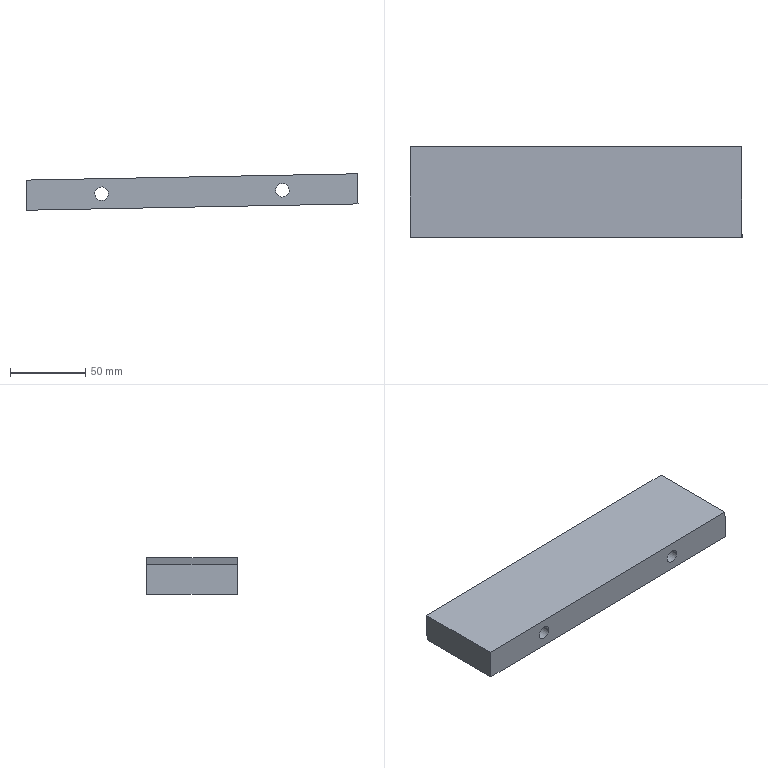Component | SolidWorks | 12TopPostMountingPlateSpacer-1 | 1 solid | 24 faces | box 220.34 x 60 x 24.19 mm | volume 248965 mm3 | cylinder 12 | plane 8 | cone 4 | commonest cylinder face diameters 15 x4 9 x4 8.5 x4 | material A3 Steel
build123d program:
from build123d import *

# Parameters (mm, degrees)
SKETCH1_W                                          = 220
SKETCH1_H                                          = 20
BOSS_EXTRUDE1_DEPTH                                = 30
M10_TAPPED_HOLE1_D                                 = 8.5
M10_TAPPED_HOLE1_DEPTH                             = 24.5
M10_TAPPED_HOLE1_TIP                               = 2.554
HOLE_SIZE_ACCORDING_TO_TYPE_1_OF_HEXAG_D           = 9
HOLE_SIZE_ACCORDING_TO_TYPE_1_OF_HEXAG_CBORE_D     = 15
HOLE_SIZE_ACCORDING_TO_TYPE_1_OF_HEXAG_CBORE_DEPTH = 20


with BuildPart() as part:
    # Sketch1 → Boss-Extrude1 (new, symmetric)
    with BuildSketch(Plane.XY):
        Rectangle(SKETCH1_W, SKETCH1_H)
    extrude(amount=BOSS_EXTRUDE1_DEPTH, both=True)

    # M10 Tapped Hole1
    with Locations(Plane(origin=(-90, 0, -30), x_dir=(-1, 0, 0), z_dir=(0, 0, -1))):
        with Locations((0, 0), (-180, 0)):
            Hole(M10_TAPPED_HOLE1_D / 2, depth=M10_TAPPED_HOLE1_DEPTH)
            with Locations((0, 0, -(M10_TAPPED_HOLE1_DEPTH + M10_TAPPED_HOLE1_TIP / 2))):  # 118° drill point
                Cone(0, M10_TAPPED_HOLE1_D / 2, M10_TAPPED_HOLE1_TIP, mode=Mode.SUBTRACT)

    # Hole Size _According to_ Type 1 of Hexag (through all)
    with Locations(Plane(origin=(60, 0, -30), x_dir=(-1, 0, 0), z_dir=(0, 0, -1))):
        with Locations((0, 0), (120, 0)):
            CounterBoreHole(HOLE_SIZE_ACCORDING_TO_TYPE_1_OF_HEXAG_D / 2, HOLE_SIZE_ACCORDING_TO_TYPE_1_OF_HEXAG_CBORE_D / 2, HOLE_SIZE_ACCORDING_TO_TYPE_1_OF_HEXAG_CBORE_DEPTH)


solid = part.part

# Placed as in the assembly
solid = solid.moved(Location((1158.199, -1865.522, 2192.697), (90, 0, 1.091)))
STEP:
#1=COLOUR_RGB('',0.7922,0.8196,0.9333);
#2=FILL_AREA_STYLE_COLOUR('',#1);
#3=FILL_AREA_STYLE('',(#2));
#4=SURFACE_STYLE_FILL_AREA(#3);
#5=SURFACE_SIDE_STYLE('',(#4));
#6=SURFACE_STYLE_USAGE(.BOTH.,#5);
#7=PRESENTATION_STYLE_ASSIGNMENT((#6));
#8=CARTESIAN_POINT('',(48.255,-73.052,86.377));
#9=VERTEX_POINT('',#8);
#10=CARTESIAN_POINT('',(47.665,-73.052,86.366));
#11=VERTEX_POINT('',#10);
#12=CARTESIAN_POINT('',(47.96,-73.052,86.372));
#13=DIRECTION('',(-0.,1.,-0.));
#14=DIRECTION('',(-0.9998,0.,-0.01904));
#15=AXIS2_PLACEMENT_3D('',#12,#13,#14);
#16=CIRCLE('',#15,0.2953);
#17=EDGE_CURVE('',#9,#11,#16,.T.);
#18=ORIENTED_EDGE('',*,*,#17,.F.);
#19=CARTESIAN_POINT('',(48.255,-72.265,86.377));
#20=VERTEX_POINT('',#19);
#21=CARTESIAN_POINT('',(48.255,-72.265,86.377));
#22=DIRECTION('',(-0.,1.,-0.));
#23=VECTOR('',#22,39.37);
#24=LINE('',#21,#23);
#25=EDGE_CURVE('',#9,#20,#24,.T.);
#26=ORIENTED_EDGE('',*,*,#25,.T.);
#27=CARTESIAN_POINT('',(47.665,-72.265,86.366));
#28=VERTEX_POINT('',#27);
#29=CARTESIAN_POINT('',(47.96,-72.265,86.372));
#30=DIRECTION('',(-0.,1.,-0.));
#31=DIRECTION('',(-0.9998,0.,-0.01904));
#32=AXIS2_PLACEMENT_3D('',#29,#30,#31);
#33=CIRCLE('',#32,0.2953);
#34=EDGE_CURVE('',#20,#28,#33,.T.);
#35=ORIENTED_EDGE('',*,*,#34,.T.);
#36=CARTESIAN_POINT('',(47.665,-72.265,86.366));
#37=DIRECTION('',(-0.,1.,-0.));
#38=VECTOR('',#37,39.37);
#39=LINE('',#36,#38);
#40=EDGE_CURVE('',#11,#28,#39,.T.);
#41=ORIENTED_EDGE('',*,*,#40,.F.);
#42=EDGE_LOOP('',(#18,#26,#35,#41));
#43=FACE_OUTER_BOUND('',#42,.T.);
#44=CARTESIAN_POINT('',(47.96,-72.265,86.372));
#45=DIRECTION('',(-0.,1.,-0.));
#46=DIRECTION('',(-0.9998,0.,-0.01904));
#47=AXIS2_PLACEMENT_3D('',#44,#45,#46);
#48=CYLINDRICAL_SURFACE('',#47,0.2953);
#49=ADVANCED_FACE('',(#43),#48,.F.);
#50=CARTESIAN_POINT('',(48.137,-74.627,86.375));
#51=VERTEX_POINT('',#50);
#52=CARTESIAN_POINT('',(47.783,-74.627,86.368));
#53=VERTEX_POINT('',#52);
#54=CARTESIAN_POINT('',(47.96,-74.627,86.372));
#55=DIRECTION('',(-0.,1.,-0.));
#56=DIRECTION('',(-0.9998,0.,-0.01904));
#57=AXIS2_PLACEMENT_3D('',#54,#55,#56);
#58=CIRCLE('',#57,0.1772);
#59=EDGE_CURVE('',#51,#53,#58,.T.);
#60=ORIENTED_EDGE('',*,*,#59,.F.);
#61=CARTESIAN_POINT('',(48.137,-73.052,86.375));
#62=VERTEX_POINT('',#61);
#63=CARTESIAN_POINT('',(48.137,-72.265,86.375));
#64=DIRECTION('',(-0.,1.,-0.));
#65=VECTOR('',#64,39.37);
#66=LINE('',#63,#65);
#67=EDGE_CURVE('',#51,#62,#66,.T.);
#68=ORIENTED_EDGE('',*,*,#67,.T.);
#69=CARTESIAN_POINT('',(47.783,-73.052,86.368));
#70=VERTEX_POINT('',#69);
#71=CARTESIAN_POINT('',(47.96,-73.052,86.372));
#72=DIRECTION('',(-0.,1.,-0.));
#73=DIRECTION('',(-0.9998,0.,-0.01904));
#74=AXIS2_PLACEMENT_3D('',#71,#72,#73);
#75=CIRCLE('',#74,0.1772);
#76=EDGE_CURVE('',#62,#70,#75,.T.);
#77=ORIENTED_EDGE('',*,*,#76,.T.);
#78=CARTESIAN_POINT('',(47.783,-72.265,86.368));
#79=DIRECTION('',(-0.,1.,-0.));
#80=VECTOR('',#79,39.37);
#81=LINE('',#78,#80);
#82=EDGE_CURVE('',#53,#70,#81,.T.);
#83=ORIENTED_EDGE('',*,*,#82,.F.);
#84=EDGE_LOOP('',(#60,#68,#77,#83));
#85=FACE_OUTER_BOUND('',#84,.T.);
#86=CARTESIAN_POINT('',(47.96,-72.265,86.372));
#87=DIRECTION('',(-0.,1.,-0.));
#88=DIRECTION('',(-0.9998,0.,-0.01904));
#89=AXIS2_PLACEMENT_3D('',#86,#87,#88);
#90=CYLINDRICAL_SURFACE('',#89,0.1772);
#91=ADVANCED_FACE('',(#85),#90,.F.);
#92=CARTESIAN_POINT('',(43.532,-73.052,86.287));
#93=VERTEX_POINT('',#92);
#94=CARTESIAN_POINT('',(42.941,-73.052,86.276));
#95=VERTEX_POINT('',#94);
#96=CARTESIAN_POINT('',(43.237,-73.052,86.282));
#97=DIRECTION('',(-0.,1.,-0.));
#98=DIRECTION('',(-0.9998,0.,-0.01904));
#99=AXIS2_PLACEMENT_3D('',#96,#97,#98);
#100=CIRCLE('',#99,0.2953);
#101=EDGE_CURVE('',#93,#95,#100,.T.);
#102=ORIENTED_EDGE('',*,*,#101,.F.);
#103=CARTESIAN_POINT('',(43.532,-72.265,86.287));
#104=VERTEX_POINT('',#103);
#105=CARTESIAN_POINT('',(43.532,-72.265,86.287));
#106=DIRECTION('',(-0.,1.,-0.));
#107=VECTOR('',#106,39.37);
#108=LINE('',#105,#107);
#109=EDGE_CURVE('',#93,#104,#108,.T.);
#110=ORIENTED_EDGE('',*,*,#109,.T.);
#111=CARTESIAN_POINT('',(42.941,-72.265,86.276));
#112=VERTEX_POINT('',#111);
#113=CARTESIAN_POINT('',(43.237,-72.265,86.282));
#114=DIRECTION('',(-0.,1.,-0.));
#115=DIRECTION('',(-0.9998,0.,-0.01904));
#116=AXIS2_PLACEMENT_3D('',#113,#114,#115);
#117=CIRCLE('',#116,0.2953);
#118=EDGE_CURVE('',#104,#112,#117,.T.);
#119=ORIENTED_EDGE('',*,*,#118,.T.);
#120=CARTESIAN_POINT('',(42.941,-72.265,86.276));
#121=DIRECTION('',(-0.,1.,-0.));
#122=VECTOR('',#121,39.37);
#123=LINE('',#120,#122);
#124=EDGE_CURVE('',#95,#112,#123,.T.);
#125=ORIENTED_EDGE('',*,*,#124,.F.);
#126=EDGE_LOOP('',(#102,#110,#119,#125));
#127=FACE_OUTER_BOUND('',#126,.T.);
#128=CARTESIAN_POINT('',(43.237,-72.265,86.282));
#129=DIRECTION('',(-0.,1.,-0.));
#130=DIRECTION('',(-0.9998,0.,-0.01904));
#131=AXIS2_PLACEMENT_3D('',#128,#129,#130);
#132=CYLINDRICAL_SURFACE('',#131,0.2953);
#133=ADVANCED_FACE('',(#127),#132,.F.);
#134=CARTESIAN_POINT('',(43.414,-74.627,86.285));
#135=VERTEX_POINT('',#134);
#136=CARTESIAN_POINT('',(43.059,-74.627,86.278));
#137=VERTEX_POINT('',#136);
#138=CARTESIAN_POINT('',(43.237,-74.627,86.282));
#139=DIRECTION('',(-0.,1.,-0.));
#140=DIRECTION('',(-0.9998,0.,-0.01904));
#141=AXIS2_PLACEMENT_3D('',#138,#139,#140);
#142=CIRCLE('',#141,0.1772);
#143=EDGE_CURVE('',#135,#137,#142,.T.);
#144=ORIENTED_EDGE('',*,*,#143,.F.);
#145=CARTESIAN_POINT('',(43.414,-73.052,86.285));
#146=VERTEX_POINT('',#145);
#147=CARTESIAN_POINT('',(43.414,-72.265,86.285));
#148=DIRECTION('',(-0.,1.,-0.));
#149=VECTOR('',#148,39.37);
#150=LINE('',#147,#149);
#151=EDGE_CURVE('',#135,#146,#150,.T.);
#152=ORIENTED_EDGE('',*,*,#151,.T.);
#153=CARTESIAN_POINT('',(43.059,-73.052,86.278));
#154=VERTEX_POINT('',#153);
#155=CARTESIAN_POINT('',(43.237,-73.052,86.282));
#156=DIRECTION('',(-0.,1.,-0.));
#157=DIRECTION('',(-0.9998,0.,-0.01904));
#158=AXIS2_PLACEMENT_3D('',#155,#156,#157);
#159=CIRCLE('',#158,0.1772);
#160=EDGE_CURVE('',#146,#154,#159,.T.);
#161=ORIENTED_EDGE('',*,*,#160,.T.);
#162=CARTESIAN_POINT('',(43.059,-72.265,86.278));
#163=DIRECTION('',(-0.,1.,-0.));
#164=VECTOR('',#163,39.37);
#165=LINE('',#162,#164);
#166=EDGE_CURVE('',#137,#154,#165,.T.);
#167=ORIENTED_EDGE('',*,*,#166,.F.);
#168=EDGE_LOOP('',(#144,#152,#161,#167));
#169=FACE_OUTER_BOUND('',#168,.T.);
#170=CARTESIAN_POINT('',(43.237,-72.265,86.282));
#171=DIRECTION('',(-0.,1.,-0.));
#172=DIRECTION('',(-0.9998,0.,-0.01904));
#173=AXIS2_PLACEMENT_3D('',#170,#171,#172);
#174=CYLINDRICAL_SURFACE('',#173,0.1772);
#175=ADVANCED_FACE('',(#169),#174,.F.);
#176=CARTESIAN_POINT('',(42.223,-73.229,86.262));
#177=VERTEX_POINT('',#176);
#178=CARTESIAN_POINT('',(41.888,-73.229,86.256));
#179=VERTEX_POINT('',#178);
#180=CARTESIAN_POINT('',(42.056,-73.229,86.259));
#181=DIRECTION('',(-0.,1.,-0.));
#182=DIRECTION('',(-0.9998,0.,-0.01904));
#183=AXIS2_PLACEMENT_3D('',#180,#181,#182);
#184=CIRCLE('',#183,0.1673);
#185=EDGE_CURVE('',#177,#179,#184,.T.);
#186=ORIENTED_EDGE('',*,*,#185,.F.);
#187=CARTESIAN_POINT('',(42.223,-72.265,86.262));
#188=VERTEX_POINT('',#187);
#189=CARTESIAN_POINT('',(42.223,-72.265,86.262));
#190=DIRECTION('',(-0.,1.,-0.));
#191=VECTOR('',#190,39.37);
#192=LINE('',#189,#191);
#193=EDGE_CURVE('',#177,#188,#192,.T.);
#194=ORIENTED_EDGE('',*,*,#193,.T.);
#195=CARTESIAN_POINT('',(41.888,-72.265,86.256));
#196=VERTEX_POINT('',#195);
#197=CARTESIAN_POINT('',(42.056,-72.265,86.259));
#198=DIRECTION('',(-0.,1.,-0.));
#199=DIRECTION('',(-0.9998,0.,-0.01904));
#200=AXIS2_PLACEMENT_3D('',#197,#198,#199);
#201=CIRCLE('',#200,0.1673);
#202=EDGE_CURVE('',#188,#196,#201,.T.);
#203=ORIENTED_EDGE('',*,*,#202,.T.);
#204=CARTESIAN_POINT('',(41.888,-72.265,86.256));
#205=DIRECTION('',(-0.,1.,-0.));
#206=VECTOR('',#205,39.37);
#207=LINE('',#204,#206);
#208=EDGE_CURVE('',#179,#196,#207,.T.);
#209=ORIENTED_EDGE('',*,*,#208,.F.);
#210=EDGE_LOOP('',(#186,#194,#203,#209));
#211=FACE_OUTER_BOUND('',#210,.T.);
#212=CARTESIAN_POINT('',(42.056,-72.265,86.259));
#213=DIRECTION('',(-0.,1.,-0.));
#214=DIRECTION('',(-0.9998,0.,-0.01904));
#215=AXIS2_PLACEMENT_3D('',#212,#213,#214);
#216=CYLINDRICAL_SURFACE('',#215,0.1673);
#217=ADVANCED_FACE('',(#211),#216,.F.);
#218=CARTESIAN_POINT('',(42.056,-73.33,86.259));
#219=VERTEX_POINT('',#218);
#220=CARTESIAN_POINT('',(41.888,-73.229,86.256));
#221=DIRECTION('',(-0.857,0.515,-0.01632));
#222=VECTOR('',#221,39.37);
#223=LINE('',#220,#222);
#224=EDGE_CURVE('',#219,#179,#223,.T.);
#225=ORIENTED_EDGE('',*,*,#224,.F.);
#226=CARTESIAN_POINT('',(42.223,-73.229,86.262));
#227=DIRECTION('',(0.857,0.515,0.01632));
#228=VECTOR('',#227,39.37);
#229=LINE('',#226,#228);
#230=EDGE_CURVE('',#219,#177,#229,.T.);
#231=ORIENTED_EDGE('',*,*,#230,.T.);
#232=ORIENTED_EDGE('',*,*,#185,.T.);
#233=EDGE_LOOP('',(#225,#231,#232));
#234=FACE_OUTER_BOUND('',#233,.T.);
#235=CARTESIAN_POINT('',(42.056,-73.229,86.259));
#236=DIRECTION('',(-0.,1.,-0.));
#237=DIRECTION('',(-0.9998,0.,-0.01904));
#238=AXIS2_PLACEMENT_3D('',#235,#236,#237);
#239=CONICAL_SURFACE('',#238,0.1673,1.03);
#240=ADVANCED_FACE('',(#234),#239,.F.);
#241=CARTESIAN_POINT('',(49.308,-73.229,86.397));
#242=VERTEX_POINT('',#241);
#243=CARTESIAN_POINT('',(48.974,-73.229,86.391));
#244=VERTEX_POINT('',#243);
#245=CARTESIAN_POINT('',(49.141,-73.229,86.394));
#246=DIRECTION('',(-0.,1.,-0.));
#247=DIRECTION('',(-0.9998,0.,-0.01904));
#248=AXIS2_PLACEMENT_3D('',#245,#246,#247);
#249=CIRCLE('',#248,0.1673);
#250=EDGE_CURVE('',#242,#244,#249,.T.);
#251=ORIENTED_EDGE('',*,*,#250,.F.);
#252=CARTESIAN_POINT('',(49.308,-72.265,86.397));
#253=VERTEX_POINT('',#252);
#254=CARTESIAN_POINT('',(49.308,-72.265,86.397));
#255=DIRECTION('',(-0.,1.,-0.));
#256=VECTOR('',#255,39.37);
#257=LINE('',#254,#256);
#258=EDGE_CURVE('',#242,#253,#257,.T.);
#259=ORIENTED_EDGE('',*,*,#258,.T.);
#260=CARTESIAN_POINT('',(48.974,-72.265,86.391));
#261=VERTEX_POINT('',#260);
#262=CARTESIAN_POINT('',(49.141,-72.265,86.394));
#263=DIRECTION('',(-0.,1.,-0.));
#264=DIRECTION('',(-0.9998,0.,-0.01904));
#265=AXIS2_PLACEMENT_3D('',#262,#263,#264);
#266=CIRCLE('',#265,0.1673);
#267=EDGE_CURVE('',#253,#261,#266,.T.);
#268=ORIENTED_EDGE('',*,*,#267,.T.);
#269=CARTESIAN_POINT('',(48.974,-72.265,86.391));
#270=DIRECTION('',(-0.,1.,-0.));
#271=VECTOR('',#270,39.37);
#272=LINE('',#269,#271);
#273=EDGE_CURVE('',#244,#261,#272,.T.);
#274=ORIENTED_EDGE('',*,*,#273,.F.);
#275=EDGE_LOOP('',(#251,#259,#268,#274));
#276=FACE_OUTER_BOUND('',#275,.T.);
#277=CARTESIAN_POINT('',(49.141,-72.265,86.394));
#278=DIRECTION('',(-0.,1.,-0.));
#279=DIRECTION('',(-0.9998,0.,-0.01904));
#280=AXIS2_PLACEMENT_3D('',#277,#278,#279);
#281=CYLINDRICAL_SURFACE('',#280,0.1673);
#282=ADVANCED_FACE('',(#276),#281,.F.);
#283=CARTESIAN_POINT('',(49.141,-73.33,86.394));
#284=VERTEX_POINT('',#283);
#285=CARTESIAN_POINT('',(48.974,-73.229,86.391));
#286=DIRECTION('',(-0.857,0.515,-0.01632));
#287=VECTOR('',#286,39.37);
#288=LINE('',#285,#287);
#289=EDGE_CURVE('',#284,#244,#288,.T.);
#290=ORIENTED_EDGE('',*,*,#289,.F.);
#291=CARTESIAN_POINT('',(49.308,-73.229,86.397));
#292=DIRECTION('',(0.857,0.515,0.01632));
#293=VECTOR('',#292,39.37);
#294=LINE('',#291,#293);
#295=EDGE_CURVE('',#284,#242,#294,.T.);
#296=ORIENTED_EDGE('',*,*,#295,.T.);
#297=ORIENTED_EDGE('',*,*,#250,.T.);
#298=EDGE_LOOP('',(#290,#296,#297));
#299=FACE_OUTER_BOUND('',#298,.T.);
#300=CARTESIAN_POINT('',(49.141,-73.229,86.394));
#301=DIRECTION('',(-0.,1.,-0.));
#302=DIRECTION('',(-0.9998,0.,-0.01904));
#303=AXIS2_PLACEMENT_3D('',#300,#301,#302);
#304=CONICAL_SURFACE('',#303,0.1673,1.03);
#305=ADVANCED_FACE('',(#299),#304,.F.);
#306=CARTESIAN_POINT('',(49.936,-72.265,86.016));
#307=VERTEX_POINT('',#306);
#308=CARTESIAN_POINT('',(49.921,-72.265,86.803));
#309=VERTEX_POINT('',#308);
#310=CARTESIAN_POINT('',(49.936,-72.265,86.016));
#311=DIRECTION('',(-0.01904,0.,0.9998));
#312=VECTOR('',#311,39.37);
#313=LINE('',#310,#312);
#314=EDGE_CURVE('',#307,#309,#313,.T.);
#315=ORIENTED_EDGE('',*,*,#314,.T.);
#316=CARTESIAN_POINT('',(49.921,-74.627,86.803));
#317=VERTEX_POINT('',#316);
#318=CARTESIAN_POINT('',(49.921,-74.627,86.803));
#319=DIRECTION('',(-0.,1.,-0.));
#320=VECTOR('',#319,39.37);
#321=LINE('',#318,#320);
#322=EDGE_CURVE('',#317,#309,#321,.T.);
#323=ORIENTED_EDGE('',*,*,#322,.F.);
#324=CARTESIAN_POINT('',(49.936,-74.627,86.016));
#325=VERTEX_POINT('',#324);
#326=CARTESIAN_POINT('',(49.936,-74.627,86.016));
#327=DIRECTION('',(-0.01904,0.,0.9998));
#328=VECTOR('',#327,39.37);
#329=LINE('',#326,#328);
#330=EDGE_CURVE('',#325,#317,#329,.T.);
#331=ORIENTED_EDGE('',*,*,#330,.F.);
#332=CARTESIAN_POINT('',(49.936,-74.627,86.016));
#333=DIRECTION('',(-0.,1.,-0.));
#334=VECTOR('',#333,39.37);
#335=LINE('',#332,#334);
#336=EDGE_CURVE('',#325,#307,#335,.T.);
#337=ORIENTED_EDGE('',*,*,#336,.T.);
#338=EDGE_LOOP('',(#315,#323,#331,#337));
#339=FACE_OUTER_BOUND('',#338,.T.);
#340=CARTESIAN_POINT('',(49.936,-74.627,86.016));
#341=DIRECTION('',(-0.9998,-0.,-0.01904));
#342=DIRECTION('',(0.,-1.,0.));
#343=AXIS2_PLACEMENT_3D('',#340,#341,#342);
#344=PLANE('',#343);
#345=ADVANCED_FACE('',(#339),#344,.F.);
#346=CARTESIAN_POINT('',(41.261,-72.265,86.638));
#347=VERTEX_POINT('',#346);
#348=CARTESIAN_POINT('',(41.261,-72.265,86.638));
#349=DIRECTION('',(-0.9998,-0.,-0.01904));
#350=VECTOR('',#349,39.37);
#351=LINE('',#348,#350);
#352=EDGE_CURVE('',#309,#347,#351,.T.);
#353=ORIENTED_EDGE('',*,*,#352,.T.);
#354=CARTESIAN_POINT('',(41.261,-74.627,86.638));
#355=VERTEX_POINT('',#354);
#356=CARTESIAN_POINT('',(41.261,-74.627,86.638));
#357=DIRECTION('',(-0.,1.,-0.));
#358=VECTOR('',#357,39.37);
#359=LINE('',#356,#358);
#360=EDGE_CURVE('',#355,#347,#359,.T.);
#361=ORIENTED_EDGE('',*,*,#360,.F.);
#362=CARTESIAN_POINT('',(41.261,-74.627,86.638));
#363=DIRECTION('',(-0.9998,-0.,-0.01904));
#364=VECTOR('',#363,39.37);
#365=LINE('',#362,#364);
#366=EDGE_CURVE('',#317,#355,#365,.T.);
#367=ORIENTED_EDGE('',*,*,#366,.F.);
#368=ORIENTED_EDGE('',*,*,#322,.T.);
#369=EDGE_LOOP('',(#353,#361,#367,#368));
#370=FACE_OUTER_BOUND('',#369,.T.);
#371=CARTESIAN_POINT('',(41.261,-74.627,86.638));
#372=DIRECTION('',(0.01904,-0.,-0.9998));
#373=DIRECTION('',(-0.,1.,-0.));
#374=AXIS2_PLACEMENT_3D('',#371,#372,#373);
#375=PLANE('',#374);
#376=ADVANCED_FACE('',(#370),#375,.F.);
#377=CARTESIAN_POINT('',(41.276,-72.265,85.851));
#378=VERTEX_POINT('',#377);
#379=CARTESIAN_POINT('',(41.276,-72.265,85.851));
#380=DIRECTION('',(0.01904,-0.,-0.9998));
#381=VECTOR('',#380,39.37);
#382=LINE('',#379,#381);
#383=EDGE_CURVE('',#347,#378,#382,.T.);
#384=ORIENTED_EDGE('',*,*,#383,.T.);
#385=CARTESIAN_POINT('',(41.276,-74.627,85.851));
#386=VERTEX_POINT('',#385);
#387=CARTESIAN_POINT('',(41.276,-74.627,85.851));
#388=DIRECTION('',(-0.,1.,-0.));
#389=VECTOR('',#388,39.37);
#390=LINE('',#387,#389);
#391=EDGE_CURVE('',#386,#378,#390,.T.);
#392=ORIENTED_EDGE('',*,*,#391,.F.);
#393=CARTESIAN_POINT('',(41.276,-74.627,85.851));
#394=DIRECTION('',(0.01904,-0.,-0.9998));
#395=VECTOR('',#394,39.37);
#396=LINE('',#393,#395);
#397=EDGE_CURVE('',#355,#386,#396,.T.);
#398=ORIENTED_EDGE('',*,*,#397,.F.);
#399=ORIENTED_EDGE('',*,*,#360,.T.);
#400=EDGE_LOOP('',(#384,#392,#398,#399));
#401=FACE_OUTER_BOUND('',#400,.T.);
#402=CARTESIAN_POINT('',(41.276,-74.627,85.851));
#403=DIRECTION('',(0.9998,0.,0.01904));
#404=DIRECTION('',(-0.,1.,-0.));
#405=AXIS2_PLACEMENT_3D('',#402,#403,#404);
#406=PLANE('',#405);
#407=ADVANCED_FACE('',(#401),#406,.F.);
#408=CARTESIAN_POINT('',(41.276,-72.265,85.851));
#409=DIRECTION('',(0.9998,0.,0.01904));
#410=VECTOR('',#409,39.37);
#411=LINE('',#408,#410);
#412=EDGE_CURVE('',#378,#307,#411,.T.);
#413=ORIENTED_EDGE('',*,*,#412,.T.);
#414=ORIENTED_EDGE('',*,*,#336,.F.);
#415=CARTESIAN_POINT('',(41.276,-74.627,85.851));
#416=DIRECTION('',(0.9998,0.,0.01904));
#417=VECTOR('',#416,39.37);
#418=LINE('',#415,#417);
#419=EDGE_CURVE('',#386,#325,#418,.T.);
#420=ORIENTED_EDGE('',*,*,#419,.F.);
#421=ORIENTED_EDGE('',*,*,#391,.T.);
#422=EDGE_LOOP('',(#413,#414,#420,#421));
#423=FACE_OUTER_BOUND('',#422,.T.);
#424=CARTESIAN_POINT('',(41.276,-74.627,85.851));
#425=DIRECTION('',(-0.01904,0.,0.9998));
#426=DIRECTION('',(0.,-1.,0.));
#427=AXIS2_PLACEMENT_3D('',#424,#425,#426);
#428=PLANE('',#427);
#429=ADVANCED_FACE('',(#423),#428,.F.);
#430=CARTESIAN_POINT('',(47.96,-74.627,86.372));
#431=DIRECTION('',(-0.,1.,-0.));
#432=DIRECTION('',(-0.9998,0.,-0.01904));
#433=AXIS2_PLACEMENT_3D('',#430,#431,#432);
#434=CIRCLE('',#433,0.1772);
#435=EDGE_CURVE('',#53,#51,#434,.T.);
#436=ORIENTED_EDGE('',*,*,#435,.T.);
#437=ORIENTED_EDGE('',*,*,#59,.T.);
#438=EDGE_LOOP('',(#436,#437));
#439=FACE_BOUND('',#438,.T.);
#440=CARTESIAN_POINT('',(43.237,-74.627,86.282));
#441=DIRECTION('',(-0.,1.,-0.));
#442=DIRECTION('',(-0.9998,0.,-0.01904));
#443=AXIS2_PLACEMENT_3D('',#440,#441,#442);
#444=CIRCLE('',#443,0.1772);
#445=EDGE_CURVE('',#137,#135,#444,.T.);
#446=ORIENTED_EDGE('',*,*,#445,.T.);
#447=ORIENTED_EDGE('',*,*,#143,.T.);
#448=EDGE_LOOP('',(#446,#447));
#449=FACE_BOUND('',#448,.T.);
#450=ORIENTED_EDGE('',*,*,#330,.T.);
#451=ORIENTED_EDGE('',*,*,#366,.T.);
#452=ORIENTED_EDGE('',*,*,#397,.T.);
#453=ORIENTED_EDGE('',*,*,#419,.T.);
#454=EDGE_LOOP('',(#450,#451,#452,#453));
#455=FACE_OUTER_BOUND('',#454,.T.);
#456=CARTESIAN_POINT('',(45.598,-74.627,86.327));
#457=DIRECTION('',(-0.,1.,-0.));
#458=DIRECTION('',(-0.9998,-0.,-0.01904));
#459=AXIS2_PLACEMENT_3D('',#456,#457,#458);
#460=PLANE('',#459);
#461=ADVANCED_FACE('',(#439,#449,#455),#460,.F.);
#462=CARTESIAN_POINT('',(47.96,-72.265,86.372));
#463=DIRECTION('',(-0.,1.,-0.));
#464=DIRECTION('',(-0.9998,0.,-0.01904));
#465=AXIS2_PLACEMENT_3D('',#462,#463,#464);
#466=CIRCLE('',#465,0.2953);
#467=EDGE_CURVE('',#28,#20,#466,.T.);
#468=ORIENTED_EDGE('',*,*,#467,.F.);
#469=ORIENTED_EDGE('',*,*,#34,.F.);
#470=EDGE_LOOP('',(#468,#469));
#471=FACE_BOUND('',#470,.T.);
#472=CARTESIAN_POINT('',(43.237,-72.265,86.282));
#473=DIRECTION('',(-0.,1.,-0.));
#474=DIRECTION('',(-0.9998,0.,-0.01904));
#475=AXIS2_PLACEMENT_3D('',#472,#473,#474);
#476=CIRCLE('',#475,0.2953);
#477=EDGE_CURVE('',#112,#104,#476,.T.);
#478=ORIENTED_EDGE('',*,*,#477,.F.);
#479=ORIENTED_EDGE('',*,*,#118,.F.);
#480=EDGE_LOOP('',(#478,#479));
#481=FACE_BOUND('',#480,.T.);
#482=CARTESIAN_POINT('',(42.056,-72.265,86.259));
#483=DIRECTION('',(-0.,1.,-0.));
#484=DIRECTION('',(-0.9998,0.,-0.01904));
#485=AXIS2_PLACEMENT_3D('',#482,#483,#484);
#486=CIRCLE('',#485,0.1673);
#487=EDGE_CURVE('',#196,#188,#486,.T.);
#488=ORIENTED_EDGE('',*,*,#487,.F.);
#489=ORIENTED_EDGE('',*,*,#202,.F.);
#490=EDGE_LOOP('',(#488,#489));
#491=FACE_BOUND('',#490,.T.);
#492=CARTESIAN_POINT('',(49.141,-72.265,86.394));
#493=DIRECTION('',(-0.,1.,-0.));
#494=DIRECTION('',(-0.9998,0.,-0.01904));
#495=AXIS2_PLACEMENT_3D('',#492,#493,#494);
#496=CIRCLE('',#495,0.1673);
#497=EDGE_CURVE('',#261,#253,#496,.T.);
#498=ORIENTED_EDGE('',*,*,#497,.F.);
#499=ORIENTED_EDGE('',*,*,#267,.F.);
#500=EDGE_LOOP('',(#498,#499));
#501=FACE_BOUND('',#500,.T.);
#502=ORIENTED_EDGE('',*,*,#314,.F.);
#503=ORIENTED_EDGE('',*,*,#412,.F.);
#504=ORIENTED_EDGE('',*,*,#383,.F.);
#505=ORIENTED_EDGE('',*,*,#352,.F.);
#506=EDGE_LOOP('',(#502,#503,#504,#505));
#507=FACE_OUTER_BOUND('',#506,.T.);
#508=CARTESIAN_POINT('',(45.598,-72.265,86.327));
#509=DIRECTION('',(-0.,1.,-0.));
#510=DIRECTION('',(-0.9998,-0.,-0.01904));
#511=AXIS2_PLACEMENT_3D('',#508,#509,#510);
#512=PLANE('',#511);
#513=ADVANCED_FACE('',(#471,#481,#491,#501,#507),#512,.T.);
#514=ORIENTED_EDGE('',*,*,#295,.F.);
#515=ORIENTED_EDGE('',*,*,#289,.T.);
#516=CARTESIAN_POINT('',(49.141,-73.229,86.394));
#517=DIRECTION('',(-0.,1.,-0.));
#518=DIRECTION('',(-0.9998,0.,-0.01904));
#519=AXIS2_PLACEMENT_3D('',#516,#517,#518);
#520=CIRCLE('',#519,0.1673);
#521=EDGE_CURVE('',#244,#242,#520,.T.);
#522=ORIENTED_EDGE('',*,*,#521,.T.);
#523=EDGE_LOOP('',(#514,#515,#522));
#524=FACE_OUTER_BOUND('',#523,.T.);
#525=CARTESIAN_POINT('',(49.141,-73.229,86.394));
#526=DIRECTION('',(-0.,1.,-0.));
#527=DIRECTION('',(-0.9998,0.,-0.01904));
#528=AXIS2_PLACEMENT_3D('',#525,#526,#527);
#529=CONICAL_SURFACE('',#528,0.1673,1.03);
#530=ADVANCED_FACE('',(#524),#529,.F.);
#531=ORIENTED_EDGE('',*,*,#258,.F.);
#532=ORIENTED_EDGE('',*,*,#521,.F.);
#533=ORIENTED_EDGE('',*,*,#273,.T.);
#534=ORIENTED_EDGE('',*,*,#497,.T.);
#535=EDGE_LOOP('',(#531,#532,#533,#534));
#536=FACE_OUTER_BOUND('',#535,.T.);
#537=CARTESIAN_POINT('',(49.141,-72.265,86.394));
#538=DIRECTION('',(-0.,1.,-0.));
#539=DIRECTION('',(-0.9998,0.,-0.01904));
#540=AXIS2_PLACEMENT_3D('',#537,#538,#539);
#541=CYLINDRICAL_SURFACE('',#540,0.1673);
#542=ADVANCED_FACE('',(#536),#541,.F.);
#543=ORIENTED_EDGE('',*,*,#230,.F.);
#544=ORIENTED_EDGE('',*,*,#224,.T.);
#545=CARTESIAN_POINT('',(42.056,-73.229,86.259));
#546=DIRECTION('',(-0.,1.,-0.));
#547=DIRECTION('',(-0.9998,0.,-0.01904));
#548=AXIS2_PLACEMENT_3D('',#545,#546,#547);
#549=CIRCLE('',#548,0.1673);
#550=EDGE_CURVE('',#179,#177,#549,.T.);
#551=ORIENTED_EDGE('',*,*,#550,.T.);
#552=EDGE_LOOP('',(#543,#544,#551));
#553=FACE_OUTER_BOUND('',#552,.T.);
#554=CARTESIAN_POINT('',(42.056,-73.229,86.259));
#555=DIRECTION('',(-0.,1.,-0.));
#556=DIRECTION('',(-0.9998,0.,-0.01904));
#557=AXIS2_PLACEMENT_3D('',#554,#555,#556);
#558=CONICAL_SURFACE('',#557,0.1673,1.03);
#559=ADVANCED_FACE('',(#553),#558,.F.);
#560=ORIENTED_EDGE('',*,*,#193,.F.);
#561=ORIENTED_EDGE('',*,*,#550,.F.);
#562=ORIENTED_EDGE('',*,*,#208,.T.);
#563=ORIENTED_EDGE('',*,*,#487,.T.);
#564=EDGE_LOOP('',(#560,#561,#562,#563));
#565=FACE_OUTER_BOUND('',#564,.T.);
#566=CARTESIAN_POINT('',(42.056,-72.265,86.259));
#567=DIRECTION('',(-0.,1.,-0.));
#568=DIRECTION('',(-0.9998,0.,-0.01904));
#569=AXIS2_PLACEMENT_3D('',#566,#567,#568);
#570=CYLINDRICAL_SURFACE('',#569,0.1673);
#571=ADVANCED_FACE('',(#565),#570,.F.);
#572=ORIENTED_EDGE('',*,*,#151,.F.);
#573=ORIENTED_EDGE('',*,*,#445,.F.);
#574=ORIENTED_EDGE('',*,*,#166,.T.);
#575=CARTESIAN_POINT('',(43.237,-73.052,86.282));
#576=DIRECTION('',(-0.,1.,-0.));
#577=DIRECTION('',(-0.9998,0.,-0.01904));
#578=AXIS2_PLACEMENT_3D('',#575,#576,#577);
#579=CIRCLE('',#578,0.1772);
#580=EDGE_CURVE('',#154,#146,#579,.T.);
#581=ORIENTED_EDGE('',*,*,#580,.T.);
#582=EDGE_LOOP('',(#572,#573,#574,#581));
#583=FACE_OUTER_BOUND('',#582,.T.);
#584=CARTESIAN_POINT('',(43.237,-72.265,86.282));
#585=DIRECTION('',(-0.,1.,-0.));
#586=DIRECTION('',(-0.9998,0.,-0.01904));
#587=AXIS2_PLACEMENT_3D('',#584,#585,#586);
#588=CYLINDRICAL_SURFACE('',#587,0.1772);
#589=ADVANCED_FACE('',(#583),#588,.F.);
#590=ORIENTED_EDGE('',*,*,#580,.F.);
#591=ORIENTED_EDGE('',*,*,#160,.F.);
#592=EDGE_LOOP('',(#590,#591));
#593=FACE_BOUND('',#592,.T.);
#594=CARTESIAN_POINT('',(43.237,-73.052,86.282));
#595=DIRECTION('',(-0.,1.,-0.));
#596=DIRECTION('',(-0.9998,0.,-0.01904));
#597=AXIS2_PLACEMENT_3D('',#594,#595,#596);
#598=CIRCLE('',#597,0.2953);
#599=EDGE_CURVE('',#95,#93,#598,.T.);
#600=ORIENTED_EDGE('',*,*,#599,.T.);
#601=ORIENTED_EDGE('',*,*,#101,.T.);
#602=EDGE_LOOP('',(#600,#601));
#603=FACE_OUTER_BOUND('',#602,.T.);
#604=CARTESIAN_POINT('',(43.414,-73.052,86.285));
#605=DIRECTION('',(0.,-1.,0.));
#606=DIRECTION('',(0.9998,0.,0.01904));
#607=AXIS2_PLACEMENT_3D('',#604,#605,#606);
#608=PLANE('',#607);
#609=ADVANCED_FACE('',(#593,#603),#608,.F.);
#610=ORIENTED_EDGE('',*,*,#109,.F.);
#611=ORIENTED_EDGE('',*,*,#599,.F.);
#612=ORIENTED_EDGE('',*,*,#124,.T.);
#613=ORIENTED_EDGE('',*,*,#477,.T.);
#614=EDGE_LOOP('',(#610,#611,#612,#613));
#615=FACE_OUTER_BOUND('',#614,.T.);
#616=CARTESIAN_POINT('',(43.237,-72.265,86.282));
#617=DIRECTION('',(-0.,1.,-0.));
#618=DIRECTION('',(-0.9998,0.,-0.01904));
#619=AXIS2_PLACEMENT_3D('',#616,#617,#618);
#620=CYLINDRICAL_SURFACE('',#619,0.2953);
#621=ADVANCED_FACE('',(#615),#620,.F.);
#622=ORIENTED_EDGE('',*,*,#67,.F.);
#623=ORIENTED_EDGE('',*,*,#435,.F.);
#624=ORIENTED_EDGE('',*,*,#82,.T.);
#625=CARTESIAN_POINT('',(47.96,-73.052,86.372));
#626=DIRECTION('',(-0.,1.,-0.));
#627=DIRECTION('',(-0.9998,0.,-0.01904));
#628=AXIS2_PLACEMENT_3D('',#625,#626,#627);
#629=CIRCLE('',#628,0.1772);
#630=EDGE_CURVE('',#70,#62,#629,.T.);
#631=ORIENTED_EDGE('',*,*,#630,.T.);
#632=EDGE_LOOP('',(#622,#623,#624,#631));
#633=FACE_OUTER_BOUND('',#632,.T.);
#634=CARTESIAN_POINT('',(47.96,-72.265,86.372));
#635=DIRECTION('',(-0.,1.,-0.));
#636=DIRECTION('',(-0.9998,0.,-0.01904));
#637=AXIS2_PLACEMENT_3D('',#634,#635,#636);
#638=CYLINDRICAL_SURFACE('',#637,0.1772);
#639=ADVANCED_FACE('',(#633),#638,.F.);
#640=ORIENTED_EDGE('',*,*,#630,.F.);
#641=ORIENTED_EDGE('',*,*,#76,.F.);
#642=EDGE_LOOP('',(#640,#641));
#643=FACE_BOUND('',#642,.T.);
#644=CARTESIAN_POINT('',(47.96,-73.052,86.372));
#645=DIRECTION('',(-0.,1.,-0.));
#646=DIRECTION('',(-0.9998,0.,-0.01904));
#647=AXIS2_PLACEMENT_3D('',#644,#645,#646);
#648=CIRCLE('',#647,0.2953);
#649=EDGE_CURVE('',#11,#9,#648,.T.);
#650=ORIENTED_EDGE('',*,*,#649,.T.);
#651=ORIENTED_EDGE('',*,*,#17,.T.);
#652=EDGE_LOOP('',(#650,#651));
#653=FACE_OUTER_BOUND('',#652,.T.);
#654=CARTESIAN_POINT('',(48.137,-73.052,86.375));
#655=DIRECTION('',(0.,-1.,0.));
#656=DIRECTION('',(0.9998,0.,0.01904));
#657=AXIS2_PLACEMENT_3D('',#654,#655,#656);
#658=PLANE('',#657);
#659=ADVANCED_FACE('',(#643,#653),#658,.F.);
#660=ORIENTED_EDGE('',*,*,#25,.F.);
#661=ORIENTED_EDGE('',*,*,#649,.F.);
#662=ORIENTED_EDGE('',*,*,#40,.T.);
#663=ORIENTED_EDGE('',*,*,#467,.T.);
#664=EDGE_LOOP('',(#660,#661,#662,#663));
#665=FACE_OUTER_BOUND('',#664,.T.);
#666=CARTESIAN_POINT('',(47.96,-72.265,86.372));
#667=DIRECTION('',(-0.,1.,-0.));
#668=DIRECTION('',(-0.9998,0.,-0.01904));
#669=AXIS2_PLACEMENT_3D('',#666,#667,#668);
#670=CYLINDRICAL_SURFACE('',#669,0.2953);
#671=ADVANCED_FACE('',(#665),#670,.F.);
#672=CLOSED_SHELL('',(#49,#91,#133,#175,#217,#240,#282,#305,#345,#376,#407,#429,#461,#513,#530,#542,#559,#571,#589,#609,#621,#639,#659,#671));
#673=MANIFOLD_SOLID_BREP('',#672);
#674=STYLED_ITEM('',(#7),#673);
#675=(LENGTH_UNIT()NAMED_UNIT(*)SI_UNIT($,.METRE.));
#676=LENGTH_MEASURE_WITH_UNIT(LENGTH_MEASURE(0.0254),#675);
#677=DIMENSIONAL_EXPONENTS(1.,0.,0.,0.,0.,0.,0.);
#678=(CONVERSION_BASED_UNIT('',#676)LENGTH_UNIT()NAMED_UNIT(#677));
#679=UNCERTAINTY_MEASURE_WITH_UNIT(LENGTH_MEASURE(0.00001),#678,'','');
#680=(NAMED_UNIT(*)PLANE_ANGLE_UNIT()SI_UNIT($,.RADIAN.));
#681=(NAMED_UNIT(*)SI_UNIT($,.STERADIAN.)SOLID_ANGLE_UNIT());
#682=(GEOMETRIC_REPRESENTATION_CONTEXT(3)GLOBAL_UNCERTAINTY_ASSIGNED_CONTEXT((#679))GLOBAL_UNIT_ASSIGNED_CONTEXT((#678,#680,#681))REPRESENTATION_CONTEXT('',''));
#683=MECHANICAL_DESIGN_GEOMETRIC_PRESENTATION_REPRESENTATION('',(#674),#682);
#684=CARTESIAN_POINT('',(0.,0.,0.));
#685=DIRECTION('',(0.,0.,1.));
#686=DIRECTION('',(1.,0.,0.));
#687=AXIS2_PLACEMENT_3D('',#684,#685,#686);
#688=(LENGTH_UNIT()NAMED_UNIT(*)SI_UNIT($,.METRE.));
#689=LENGTH_MEASURE_WITH_UNIT(LENGTH_MEASURE(0.0254),#688);
#690=DIMENSIONAL_EXPONENTS(1.,0.,0.,0.,0.,0.,0.);
#691=(CONVERSION_BASED_UNIT('',#689)LENGTH_UNIT()NAMED_UNIT(#690));
#692=UNCERTAINTY_MEASURE_WITH_UNIT(LENGTH_MEASURE(0.00001),#691,'','');
#693=(NAMED_UNIT(*)PLANE_ANGLE_UNIT()SI_UNIT($,.RADIAN.));
#694=(NAMED_UNIT(*)SI_UNIT($,.STERADIAN.)SOLID_ANGLE_UNIT());
#695=(GEOMETRIC_REPRESENTATION_CONTEXT(3)GLOBAL_UNCERTAINTY_ASSIGNED_CONTEXT((#692))GLOBAL_UNIT_ASSIGNED_CONTEXT((#691,#693,#694))REPRESENTATION_CONTEXT('',''));
#696=ADVANCED_BREP_SHAPE_REPRESENTATION('',(#673,#687),#695);
#697=PRESENTATION_LAYER_ASSIGNMENT('','',(#674));